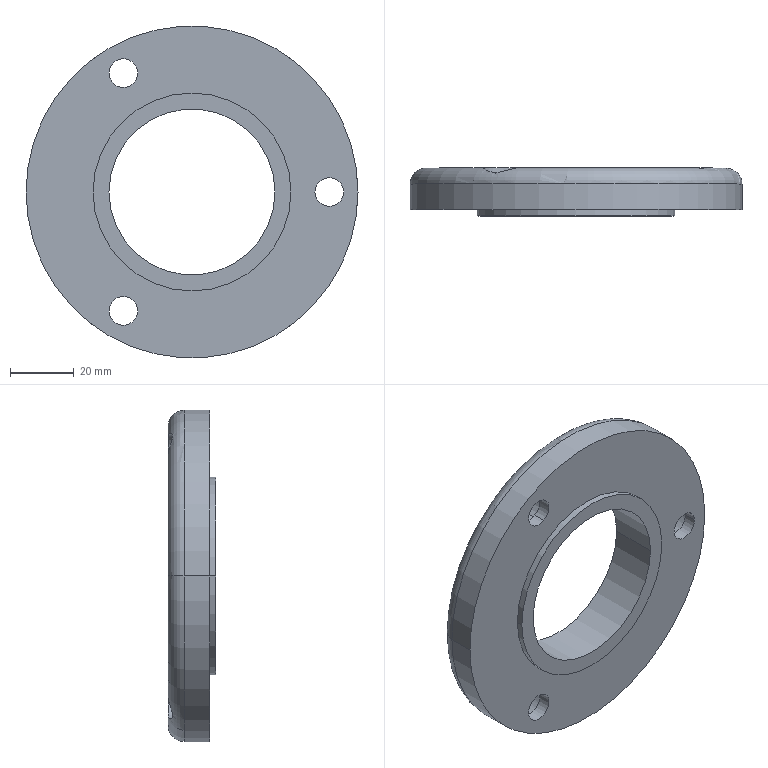Component | SolidWorks | 16-1 | 1 solid | 26 faces | box 104 x 15 x 104 mm | volume 77397 mm3 | cylinder 18 | plane 6 | torus 2 | commonest cylinder face diameters 15 x6 9 x6 52 x2 62 x2 104 x2
STEP:
#1=COLOUR_RGB('',0.7922,0.8196,0.9333);
#2=FILL_AREA_STYLE_COLOUR('',#1);
#3=FILL_AREA_STYLE('',(#2));
#4=SURFACE_STYLE_FILL_AREA(#3);
#5=SURFACE_SIDE_STYLE('',(#4));
#6=SURFACE_STYLE_USAGE(.BOTH.,#5);
#7=PRESENTATION_STYLE_ASSIGNMENT((#6));
#8=CARTESIAN_POINT('',(-1.85,-2.835,0.));
#9=VERTEX_POINT('',#8);
#10=CARTESIAN_POINT('',(-1.142,-2.835,1.456));
#11=VERTEX_POINT('',#10);
#12=CARTESIAN_POINT('',(0.,-2.835,-0.));
#13=DIRECTION('',(-0.,1.,0.));
#14=DIRECTION('',(1.,0.,0.));
#15=AXIS2_PLACEMENT_3D('',#12,#13,#14);
#16=CIRCLE('',#15,1.85);
#17=EDGE_CURVE('',#9,#11,#16,.T.);
#18=ORIENTED_EDGE('',*,*,#17,.F.);
#19=CARTESIAN_POINT('',(-2.047,-3.031,0.));
#20=VERTEX_POINT('',#19);
#21=CARTESIAN_POINT('',(-1.85,-3.031,0.));
#22=DIRECTION('',(0.,-0.,1.));
#23=DIRECTION('',(1.,0.,-0.));
#24=AXIS2_PLACEMENT_3D('',#21,#22,#23);
#25=CIRCLE('',#24,0.1969);
#26=EDGE_CURVE('',#9,#20,#25,.T.);
#27=ORIENTED_EDGE('',*,*,#26,.T.);
#28=CARTESIAN_POINT('',(2.047,-3.031,-0.));
#29=VERTEX_POINT('',#28);
#30=CARTESIAN_POINT('',(0.,-3.031,-0.));
#31=DIRECTION('',(0.,-1.,-0.));
#32=DIRECTION('',(1.,0.,-0.));
#33=AXIS2_PLACEMENT_3D('',#30,#31,#32);
#34=CIRCLE('',#33,2.047);
#35=EDGE_CURVE('',#29,#20,#34,.T.);
#36=ORIENTED_EDGE('',*,*,#35,.F.);
#37=CARTESIAN_POINT('',(1.988,-2.891,-0.));
#38=VERTEX_POINT('',#37);
#39=CARTESIAN_POINT('',(1.85,-3.031,-0.));
#40=DIRECTION('',(-0.,0.,-1.));
#41=DIRECTION('',(-1.,0.,0.));
#42=AXIS2_PLACEMENT_3D('',#39,#40,#41);
#43=CIRCLE('',#42,0.1969);
#44=EDGE_CURVE('',#38,#29,#43,.T.);
#45=ORIENTED_EDGE('',*,*,#44,.F.);
#46=CARTESIAN_POINT('',(1.832,-2.835,0.2605));
#47=VERTEX_POINT('',#46);
#48=CARTESIAN_POINT('',(1.832,-2.835,0.2605));
#49=CARTESIAN_POINT('',(1.856,-2.835,0.2476));
#50=CARTESIAN_POINT('',(1.878,-2.838,0.2318));
#51=CARTESIAN_POINT('',(1.907,-2.846,0.204));
#52=CARTESIAN_POINT('',(1.916,-2.849,0.1943));
#53=CARTESIAN_POINT('',(1.932,-2.856,0.1738));
#54=CARTESIAN_POINT('',(1.939,-2.859,0.1631));
#55=CARTESIAN_POINT('',(1.953,-2.866,0.1407));
#56=CARTESIAN_POINT('',(1.959,-2.87,0.1289));
#57=CARTESIAN_POINT('',(1.969,-2.877,0.1048));
#58=CARTESIAN_POINT('',(1.974,-2.88,0.09241));
#59=CARTESIAN_POINT('',(1.981,-2.885,0.06703));
#60=CARTESIAN_POINT('',(1.984,-2.887,0.054));
#61=CARTESIAN_POINT('',(1.987,-2.89,0.02716));
#62=CARTESIAN_POINT('',(1.988,-2.891,0.01351));
#63=CARTESIAN_POINT('',(1.988,-2.891,-0.));
#64=B_SPLINE_CURVE_WITH_KNOTS('',3,(#48,#49,#50,#51,#52,#53,#54,#55,#56,#57,#58,#59,#60,#61,#62,#63),.UNSPECIFIED.,.F.,.F.,(4,2,2,2,2,2,2,4),(0.,0.002055,0.003083,0.004111,0.005138,0.006166,0.007194,0.008222),.UNSPECIFIED.);
#65=EDGE_CURVE('',#47,#38,#64,.T.);
#66=ORIENTED_EDGE('',*,*,#65,.F.);
#67=CARTESIAN_POINT('',(-0.6904,-2.835,1.717));
#68=VERTEX_POINT('',#67);
#69=CARTESIAN_POINT('',(0.,-2.835,-0.));
#70=DIRECTION('',(-0.,1.,0.));
#71=DIRECTION('',(1.,0.,-0.));
#72=AXIS2_PLACEMENT_3D('',#69,#70,#71);
#73=CIRCLE('',#72,1.85);
#74=EDGE_CURVE('',#68,#47,#73,.T.);
#75=ORIENTED_EDGE('',*,*,#74,.F.);
#76=CARTESIAN_POINT('',(-0.9941,-2.891,1.722));
#77=VERTEX_POINT('',#76);
#78=CARTESIAN_POINT('',(-0.9941,-2.891,1.722));
#79=CARTESIAN_POINT('',(-0.9824,-2.891,1.729));
#80=CARTESIAN_POINT('',(-0.9703,-2.89,1.734));
#81=CARTESIAN_POINT('',(-0.9453,-2.887,1.745));
#82=CARTESIAN_POINT('',(-0.9325,-2.885,1.749));
#83=CARTESIAN_POINT('',(-0.894,-2.877,1.759));
#84=CARTESIAN_POINT('',(-0.8676,-2.87,1.762));
#85=CARTESIAN_POINT('',(-0.8286,-2.859,1.761));
#86=CARTESIAN_POINT('',(-0.8156,-2.856,1.76));
#87=CARTESIAN_POINT('',(-0.7896,-2.849,1.756));
#88=CARTESIAN_POINT('',(-0.7766,-2.846,1.753));
#89=CARTESIAN_POINT('',(-0.7512,-2.841,1.746));
#90=CARTESIAN_POINT('',(-0.7387,-2.839,1.741));
#91=CARTESIAN_POINT('',(-0.7141,-2.836,1.73));
#92=CARTESIAN_POINT('',(-0.702,-2.835,1.724));
#93=CARTESIAN_POINT('',(-0.6904,-2.835,1.717));
#94=B_SPLINE_CURVE_WITH_KNOTS('',3,(#78,#79,#80,#81,#82,#83,#84,#85,#86,#87,#88,#89,#90,#91,#92,#93),.UNSPECIFIED.,.F.,.F.,(4,2,2,2,2,2,2,4),(0.008222,0.009245,0.01027,0.01232,0.01334,0.01436,0.01539,0.01641),.UNSPECIFIED.);
#95=EDGE_CURVE('',#77,#68,#94,.T.);
#96=ORIENTED_EDGE('',*,*,#95,.F.);
#97=CARTESIAN_POINT('',(-1.142,-2.835,1.456));
#98=CARTESIAN_POINT('',(-1.142,-2.835,1.484));
#99=CARTESIAN_POINT('',(-1.14,-2.838,1.51));
#100=CARTESIAN_POINT('',(-1.13,-2.846,1.549));
#101=CARTESIAN_POINT('',(-1.126,-2.849,1.562));
#102=CARTESIAN_POINT('',(-1.117,-2.856,1.586));
#103=CARTESIAN_POINT('',(-1.111,-2.859,1.598));
#104=CARTESIAN_POINT('',(-1.098,-2.866,1.621));
#105=CARTESIAN_POINT('',(-1.091,-2.87,1.632));
#106=CARTESIAN_POINT('',(-1.075,-2.877,1.653));
#107=CARTESIAN_POINT('',(-1.067,-2.88,1.663));
#108=CARTESIAN_POINT('',(-1.048,-2.885,1.682));
#109=CARTESIAN_POINT('',(-1.039,-2.887,1.691));
#110=CARTESIAN_POINT('',(-1.017,-2.89,1.707));
#111=CARTESIAN_POINT('',(-1.006,-2.891,1.715));
#112=CARTESIAN_POINT('',(-0.9941,-2.891,1.722));
#113=B_SPLINE_CURVE_WITH_KNOTS('',3,(#97,#98,#99,#100,#101,#102,#103,#104,#105,#106,#107,#108,#109,#110,#111,#112),.UNSPECIFIED.,.F.,.F.,(4,2,2,2,2,2,2,4),(0.,0.002055,0.003083,0.004111,0.005138,0.006166,0.007194,0.008222),.UNSPECIFIED.);
#114=EDGE_CURVE('',#11,#77,#113,.T.);
#115=ORIENTED_EDGE('',*,*,#114,.F.);
#116=EDGE_LOOP('',(#18,#27,#36,#45,#66,#75,#96,#115));
#117=FACE_OUTER_BOUND('',#116,.T.);
#118=CARTESIAN_POINT('',(0.,-3.031,-0.));
#119=DIRECTION('',(0.,-1.,-0.));
#120=DIRECTION('',(1.,0.,-0.));
#121=AXIS2_PLACEMENT_3D('',#118,#119,#120);
#122=TOROIDAL_SURFACE('',#121,1.85,0.1969);
#123=ADVANCED_FACE('',(#117),#122,.T.);
#124=CARTESIAN_POINT('',(-0.9941,-3.189,1.722));
#125=VERTEX_POINT('',#124);
#126=CARTESIAN_POINT('',(-0.6988,-3.189,1.21));
#127=VERTEX_POINT('',#126);
#128=CARTESIAN_POINT('',(-0.8465,-3.189,1.466));
#129=DIRECTION('',(-0.,1.,0.));
#130=DIRECTION('',(0.5,0.,-0.866));
#131=AXIS2_PLACEMENT_3D('',#128,#129,#130);
#132=CIRCLE('',#131,0.2953);
#133=EDGE_CURVE('',#125,#127,#132,.T.);
#134=ORIENTED_EDGE('',*,*,#133,.F.);
#135=CARTESIAN_POINT('',(-0.9941,-2.835,1.722));
#136=DIRECTION('',(-0.,1.,0.));
#137=VECTOR('',#136,39.37);
#138=LINE('',#135,#137);
#139=EDGE_CURVE('',#125,#77,#138,.T.);
#140=ORIENTED_EDGE('',*,*,#139,.T.);
#141=ORIENTED_EDGE('',*,*,#95,.T.);
#142=CARTESIAN_POINT('',(-0.6988,-2.835,1.21));
#143=VERTEX_POINT('',#142);
#144=CARTESIAN_POINT('',(-0.8465,-2.835,1.466));
#145=DIRECTION('',(-0.,1.,0.));
#146=DIRECTION('',(0.5,0.,-0.866));
#147=AXIS2_PLACEMENT_3D('',#144,#145,#146);
#148=CIRCLE('',#147,0.2953);
#149=EDGE_CURVE('',#68,#143,#148,.T.);
#150=ORIENTED_EDGE('',*,*,#149,.T.);
#151=CARTESIAN_POINT('',(-0.6988,-2.835,1.21));
#152=DIRECTION('',(-0.,1.,0.));
#153=VECTOR('',#152,39.37);
#154=LINE('',#151,#153);
#155=EDGE_CURVE('',#127,#143,#154,.T.);
#156=ORIENTED_EDGE('',*,*,#155,.F.);
#157=EDGE_LOOP('',(#134,#140,#141,#150,#156));
#158=FACE_OUTER_BOUND('',#157,.T.);
#159=CARTESIAN_POINT('',(-0.8465,-2.835,1.466));
#160=DIRECTION('',(-0.,1.,0.));
#161=DIRECTION('',(0.5,0.,-0.866));
#162=AXIS2_PLACEMENT_3D('',#159,#160,#161);
#163=CYLINDRICAL_SURFACE('',#162,0.2953);
#164=ADVANCED_FACE('',(#158),#163,.F.);
#165=CARTESIAN_POINT('',(-0.7579,-3.346,1.313));
#166=VERTEX_POINT('',#165);
#167=CARTESIAN_POINT('',(-0.935,-3.346,1.62));
#168=VERTEX_POINT('',#167);
#169=CARTESIAN_POINT('',(-0.8465,-3.346,1.466));
#170=DIRECTION('',(0.,-1.,-0.));
#171=DIRECTION('',(-0.5,0.,0.866));
#172=AXIS2_PLACEMENT_3D('',#169,#170,#171);
#173=CIRCLE('',#172,0.1772);
#174=EDGE_CURVE('',#166,#168,#173,.T.);
#175=ORIENTED_EDGE('',*,*,#174,.T.);
#176=CARTESIAN_POINT('',(-0.935,-3.189,1.62));
#177=VERTEX_POINT('',#176);
#178=CARTESIAN_POINT('',(-0.935,-2.835,1.62));
#179=DIRECTION('',(-0.,1.,0.));
#180=VECTOR('',#179,39.37);
#181=LINE('',#178,#180);
#182=EDGE_CURVE('',#168,#177,#181,.T.);
#183=ORIENTED_EDGE('',*,*,#182,.T.);
#184=CARTESIAN_POINT('',(-0.7579,-3.189,1.313));
#185=VERTEX_POINT('',#184);
#186=CARTESIAN_POINT('',(-0.8465,-3.189,1.466));
#187=DIRECTION('',(-0.,1.,0.));
#188=DIRECTION('',(0.5,0.,-0.866));
#189=AXIS2_PLACEMENT_3D('',#186,#187,#188);
#190=CIRCLE('',#189,0.1772);
#191=EDGE_CURVE('',#177,#185,#190,.T.);
#192=ORIENTED_EDGE('',*,*,#191,.T.);
#193=CARTESIAN_POINT('',(-0.7579,-2.835,1.313));
#194=DIRECTION('',(-0.,1.,0.));
#195=VECTOR('',#194,39.37);
#196=LINE('',#193,#195);
#197=EDGE_CURVE('',#166,#185,#196,.T.);
#198=ORIENTED_EDGE('',*,*,#197,.F.);
#199=EDGE_LOOP('',(#175,#183,#192,#198));
#200=FACE_OUTER_BOUND('',#199,.T.);
#201=CARTESIAN_POINT('',(-0.8465,-2.835,1.466));
#202=DIRECTION('',(-0.,1.,0.));
#203=DIRECTION('',(0.5,0.,-0.866));
#204=AXIS2_PLACEMENT_3D('',#201,#202,#203);
#205=CYLINDRICAL_SURFACE('',#204,0.1772);
#206=ADVANCED_FACE('',(#200),#205,.F.);
#207=CARTESIAN_POINT('',(-0.9941,-3.189,-1.722));
#208=VERTEX_POINT('',#207);
#209=CARTESIAN_POINT('',(-0.6988,-3.189,-1.21));
#210=VERTEX_POINT('',#209);
#211=CARTESIAN_POINT('',(-0.8465,-3.189,-1.466));
#212=DIRECTION('',(-0.,1.,0.));
#213=DIRECTION('',(0.5,0.,0.866));
#214=AXIS2_PLACEMENT_3D('',#211,#212,#213);
#215=CIRCLE('',#214,0.2953);
#216=EDGE_CURVE('',#208,#210,#215,.T.);
#217=ORIENTED_EDGE('',*,*,#216,.F.);
#218=CARTESIAN_POINT('',(-0.9941,-2.891,-1.722));
#219=VERTEX_POINT('',#218);
#220=CARTESIAN_POINT('',(-0.9941,-2.835,-1.722));
#221=DIRECTION('',(-0.,1.,0.));
#222=VECTOR('',#221,39.37);
#223=LINE('',#220,#222);
#224=EDGE_CURVE('',#208,#219,#223,.T.);
#225=ORIENTED_EDGE('',*,*,#224,.T.);
#226=CARTESIAN_POINT('',(-1.142,-2.835,-1.456));
#227=VERTEX_POINT('',#226);
#228=CARTESIAN_POINT('',(-0.9941,-2.891,-1.722));
#229=CARTESIAN_POINT('',(-1.006,-2.891,-1.715));
#230=CARTESIAN_POINT('',(-1.017,-2.89,-1.708));
#231=CARTESIAN_POINT('',(-1.038,-2.887,-1.691));
#232=CARTESIAN_POINT('',(-1.048,-2.885,-1.682));
#233=CARTESIAN_POINT('',(-1.076,-2.877,-1.654));
#234=CARTESIAN_POINT('',(-1.092,-2.87,-1.632));
#235=CARTESIAN_POINT('',(-1.111,-2.859,-1.598));
#236=CARTESIAN_POINT('',(-1.116,-2.856,-1.586));
#237=CARTESIAN_POINT('',(-1.126,-2.849,-1.562));
#238=CARTESIAN_POINT('',(-1.13,-2.846,-1.549));
#239=CARTESIAN_POINT('',(-1.136,-2.841,-1.523));
#240=CARTESIAN_POINT('',(-1.139,-2.839,-1.51));
#241=CARTESIAN_POINT('',(-1.142,-2.836,-1.484));
#242=CARTESIAN_POINT('',(-1.142,-2.835,-1.47));
#243=CARTESIAN_POINT('',(-1.142,-2.835,-1.456));
#244=B_SPLINE_CURVE_WITH_KNOTS('',3,(#228,#229,#230,#231,#232,#233,#234,#235,#236,#237,#238,#239,#240,#241,#242,#243),.UNSPECIFIED.,.F.,.F.,(4,2,2,2,2,2,2,4),(0.008222,0.009245,0.01027,0.01232,0.01334,0.01436,0.01539,0.01641),.UNSPECIFIED.);
#245=EDGE_CURVE('',#219,#227,#244,.T.);
#246=ORIENTED_EDGE('',*,*,#245,.T.);
#247=CARTESIAN_POINT('',(-0.6988,-2.835,-1.21));
#248=VERTEX_POINT('',#247);
#249=CARTESIAN_POINT('',(-0.8465,-2.835,-1.466));
#250=DIRECTION('',(-0.,1.,0.));
#251=DIRECTION('',(0.5,0.,0.866));
#252=AXIS2_PLACEMENT_3D('',#249,#250,#251);
#253=CIRCLE('',#252,0.2953);
#254=EDGE_CURVE('',#227,#248,#253,.T.);
#255=ORIENTED_EDGE('',*,*,#254,.T.);
#256=CARTESIAN_POINT('',(-0.6988,-2.835,-1.21));
#257=DIRECTION('',(-0.,1.,0.));
#258=VECTOR('',#257,39.37);
#259=LINE('',#256,#258);
#260=EDGE_CURVE('',#210,#248,#259,.T.);
#261=ORIENTED_EDGE('',*,*,#260,.F.);
#262=EDGE_LOOP('',(#217,#225,#246,#255,#261));
#263=FACE_OUTER_BOUND('',#262,.T.);
#264=CARTESIAN_POINT('',(-0.8465,-2.835,-1.466));
#265=DIRECTION('',(-0.,1.,0.));
#266=DIRECTION('',(0.5,0.,0.866));
#267=AXIS2_PLACEMENT_3D('',#264,#265,#266);
#268=CYLINDRICAL_SURFACE('',#267,0.2953);
#269=ADVANCED_FACE('',(#263),#268,.F.);
#270=CARTESIAN_POINT('',(-0.7579,-3.346,-1.313));
#271=VERTEX_POINT('',#270);
#272=CARTESIAN_POINT('',(-0.935,-3.346,-1.62));
#273=VERTEX_POINT('',#272);
#274=CARTESIAN_POINT('',(-0.8465,-3.346,-1.466));
#275=DIRECTION('',(0.,-1.,-0.));
#276=DIRECTION('',(-0.5,0.,-0.866));
#277=AXIS2_PLACEMENT_3D('',#274,#275,#276);
#278=CIRCLE('',#277,0.1772);
#279=EDGE_CURVE('',#271,#273,#278,.T.);
#280=ORIENTED_EDGE('',*,*,#279,.T.);
#281=CARTESIAN_POINT('',(-0.935,-3.189,-1.62));
#282=VERTEX_POINT('',#281);
#283=CARTESIAN_POINT('',(-0.935,-2.835,-1.62));
#284=DIRECTION('',(-0.,1.,0.));
#285=VECTOR('',#284,39.37);
#286=LINE('',#283,#285);
#287=EDGE_CURVE('',#273,#282,#286,.T.);
#288=ORIENTED_EDGE('',*,*,#287,.T.);
#289=CARTESIAN_POINT('',(-0.7579,-3.189,-1.313));
#290=VERTEX_POINT('',#289);
#291=CARTESIAN_POINT('',(-0.8465,-3.189,-1.466));
#292=DIRECTION('',(-0.,1.,0.));
#293=DIRECTION('',(0.5,0.,0.866));
#294=AXIS2_PLACEMENT_3D('',#291,#292,#293);
#295=CIRCLE('',#294,0.1772);
#296=EDGE_CURVE('',#282,#290,#295,.T.);
#297=ORIENTED_EDGE('',*,*,#296,.T.);
#298=CARTESIAN_POINT('',(-0.7579,-2.835,-1.313));
#299=DIRECTION('',(-0.,1.,0.));
#300=VECTOR('',#299,39.37);
#301=LINE('',#298,#300);
#302=EDGE_CURVE('',#271,#290,#301,.T.);
#303=ORIENTED_EDGE('',*,*,#302,.F.);
#304=EDGE_LOOP('',(#280,#288,#297,#303));
#305=FACE_OUTER_BOUND('',#304,.T.);
#306=CARTESIAN_POINT('',(-0.8465,-2.835,-1.466));
#307=DIRECTION('',(-0.,1.,0.));
#308=DIRECTION('',(0.5,0.,0.866));
#309=AXIS2_PLACEMENT_3D('',#306,#307,#308);
#310=CYLINDRICAL_SURFACE('',#309,0.1772);
#311=ADVANCED_FACE('',(#305),#310,.F.);
#312=CARTESIAN_POINT('',(1.988,-3.189,-0.));
#313=VERTEX_POINT('',#312);
#314=CARTESIAN_POINT('',(1.398,-3.189,-0.));
#315=VERTEX_POINT('',#314);
#316=CARTESIAN_POINT('',(1.693,-3.189,-0.));
#317=DIRECTION('',(-0.,1.,0.));
#318=DIRECTION('',(-1.,0.,0.));
#319=AXIS2_PLACEMENT_3D('',#316,#317,#318);
#320=CIRCLE('',#319,0.2953);
#321=EDGE_CURVE('',#313,#315,#320,.T.);
#322=ORIENTED_EDGE('',*,*,#321,.F.);
#323=CARTESIAN_POINT('',(1.988,-2.835,-0.));
#324=DIRECTION('',(-0.,1.,0.));
#325=VECTOR('',#324,39.37);
#326=LINE('',#323,#325);
#327=EDGE_CURVE('',#313,#38,#326,.T.);
#328=ORIENTED_EDGE('',*,*,#327,.T.);
#329=CARTESIAN_POINT('',(1.832,-2.835,-0.2605));
#330=VERTEX_POINT('',#329);
#331=CARTESIAN_POINT('',(1.988,-2.891,-0.));
#332=CARTESIAN_POINT('',(1.988,-2.891,-0.01346));
#333=CARTESIAN_POINT('',(1.987,-2.89,-0.02689));
#334=CARTESIAN_POINT('',(1.984,-2.887,-0.0537));
#335=CARTESIAN_POINT('',(1.981,-2.885,-0.06684));
#336=CARTESIAN_POINT('',(1.97,-2.877,-0.1051));
#337=CARTESIAN_POINT('',(1.96,-2.87,-0.1295));
#338=CARTESIAN_POINT('',(1.939,-2.859,-0.163));
#339=CARTESIAN_POINT('',(1.932,-2.856,-0.1737));
#340=CARTESIAN_POINT('',(1.916,-2.849,-0.1943));
#341=CARTESIAN_POINT('',(1.907,-2.846,-0.2041));
#342=CARTESIAN_POINT('',(1.888,-2.841,-0.2224));
#343=CARTESIAN_POINT('',(1.877,-2.839,-0.231));
#344=CARTESIAN_POINT('',(1.856,-2.836,-0.2468));
#345=CARTESIAN_POINT('',(1.844,-2.835,-0.254));
#346=CARTESIAN_POINT('',(1.832,-2.835,-0.2605));
#347=B_SPLINE_CURVE_WITH_KNOTS('',3,(#331,#332,#333,#334,#335,#336,#337,#338,#339,#340,#341,#342,#343,#344,#345,#346),.UNSPECIFIED.,.F.,.F.,(4,2,2,2,2,2,2,4),(0.008222,0.009245,0.01027,0.01232,0.01334,0.01436,0.01539,0.01641),.UNSPECIFIED.);
#348=EDGE_CURVE('',#38,#330,#347,.T.);
#349=ORIENTED_EDGE('',*,*,#348,.T.);
#350=CARTESIAN_POINT('',(1.398,-2.835,-0.));
#351=VERTEX_POINT('',#350);
#352=CARTESIAN_POINT('',(1.693,-2.835,-0.));
#353=DIRECTION('',(-0.,1.,0.));
#354=DIRECTION('',(-1.,0.,0.));
#355=AXIS2_PLACEMENT_3D('',#352,#353,#354);
#356=CIRCLE('',#355,0.2953);
#357=EDGE_CURVE('',#330,#351,#356,.T.);
#358=ORIENTED_EDGE('',*,*,#357,.T.);
#359=CARTESIAN_POINT('',(1.398,-2.835,-0.));
#360=DIRECTION('',(-0.,1.,0.));
#361=VECTOR('',#360,39.37);
#362=LINE('',#359,#361);
#363=EDGE_CURVE('',#315,#351,#362,.T.);
#364=ORIENTED_EDGE('',*,*,#363,.F.);
#365=EDGE_LOOP('',(#322,#328,#349,#358,#364));
#366=FACE_OUTER_BOUND('',#365,.T.);
#367=CARTESIAN_POINT('',(1.693,-2.835,-0.));
#368=DIRECTION('',(-0.,1.,0.));
#369=DIRECTION('',(-1.,0.,0.));
#370=AXIS2_PLACEMENT_3D('',#367,#368,#369);
#371=CYLINDRICAL_SURFACE('',#370,0.2953);
#372=ADVANCED_FACE('',(#366),#371,.F.);
#373=CARTESIAN_POINT('',(1.516,-3.346,-0.));
#374=VERTEX_POINT('',#373);
#375=CARTESIAN_POINT('',(1.87,-3.346,-0.));
#376=VERTEX_POINT('',#375);
#377=CARTESIAN_POINT('',(1.693,-3.346,-0.));
#378=DIRECTION('',(0.,-1.,-0.));
#379=DIRECTION('',(1.,0.,-0.));
#380=AXIS2_PLACEMENT_3D('',#377,#378,#379);
#381=CIRCLE('',#380,0.1772);
#382=EDGE_CURVE('',#374,#376,#381,.T.);
#383=ORIENTED_EDGE('',*,*,#382,.T.);
#384=CARTESIAN_POINT('',(1.87,-3.189,-0.));
#385=VERTEX_POINT('',#384);
#386=CARTESIAN_POINT('',(1.87,-2.835,-0.));
#387=DIRECTION('',(-0.,1.,0.));
#388=VECTOR('',#387,39.37);
#389=LINE('',#386,#388);
#390=EDGE_CURVE('',#376,#385,#389,.T.);
#391=ORIENTED_EDGE('',*,*,#390,.T.);
#392=CARTESIAN_POINT('',(1.516,-3.189,-0.));
#393=VERTEX_POINT('',#392);
#394=CARTESIAN_POINT('',(1.693,-3.189,-0.));
#395=DIRECTION('',(-0.,1.,0.));
#396=DIRECTION('',(-1.,0.,0.));
#397=AXIS2_PLACEMENT_3D('',#394,#395,#396);
#398=CIRCLE('',#397,0.1772);
#399=EDGE_CURVE('',#385,#393,#398,.T.);
#400=ORIENTED_EDGE('',*,*,#399,.T.);
#401=CARTESIAN_POINT('',(1.516,-2.835,-0.));
#402=DIRECTION('',(-0.,1.,0.));
#403=VECTOR('',#402,39.37);
#404=LINE('',#401,#403);
#405=EDGE_CURVE('',#374,#393,#404,.T.);
#406=ORIENTED_EDGE('',*,*,#405,.F.);
#407=EDGE_LOOP('',(#383,#391,#400,#406));
#408=FACE_OUTER_BOUND('',#407,.T.);
#409=CARTESIAN_POINT('',(1.693,-2.835,-0.));
#410=DIRECTION('',(-0.,1.,0.));
#411=DIRECTION('',(-1.,0.,0.));
#412=AXIS2_PLACEMENT_3D('',#409,#410,#411);
#413=CYLINDRICAL_SURFACE('',#412,0.1772);
#414=ADVANCED_FACE('',(#408),#413,.F.);
#415=CARTESIAN_POINT('',(-1.024,-2.835,-0.));
#416=VERTEX_POINT('',#415);
#417=CARTESIAN_POINT('',(1.024,-2.835,-0.));
#418=VERTEX_POINT('',#417);
#419=CARTESIAN_POINT('',(0.,-2.835,-0.));
#420=DIRECTION('',(0.,-1.,-0.));
#421=DIRECTION('',(1.,0.,-0.));
#422=AXIS2_PLACEMENT_3D('',#419,#420,#421);
#423=CIRCLE('',#422,1.024);
#424=EDGE_CURVE('',#416,#418,#423,.T.);
#425=ORIENTED_EDGE('',*,*,#424,.F.);
#426=CARTESIAN_POINT('',(-1.024,-3.425,-0.));
#427=VERTEX_POINT('',#426);
#428=CARTESIAN_POINT('',(-1.024,-1.85,-0.));
#429=DIRECTION('',(0.,-1.,-0.));
#430=VECTOR('',#429,39.37);
#431=LINE('',#428,#430);
#432=EDGE_CURVE('',#416,#427,#431,.T.);
#433=ORIENTED_EDGE('',*,*,#432,.T.);
#434=CARTESIAN_POINT('',(1.024,-3.425,-0.));
#435=VERTEX_POINT('',#434);
#436=CARTESIAN_POINT('',(0.,-3.425,-0.));
#437=DIRECTION('',(0.,-1.,-0.));
#438=DIRECTION('',(1.,0.,-0.));
#439=AXIS2_PLACEMENT_3D('',#436,#437,#438);
#440=CIRCLE('',#439,1.024);
#441=EDGE_CURVE('',#427,#435,#440,.T.);
#442=ORIENTED_EDGE('',*,*,#441,.T.);
#443=CARTESIAN_POINT('',(1.024,-1.85,-0.));
#444=DIRECTION('',(0.,-1.,-0.));
#445=VECTOR('',#444,39.37);
#446=LINE('',#443,#445);
#447=EDGE_CURVE('',#418,#435,#446,.T.);
#448=ORIENTED_EDGE('',*,*,#447,.F.);
#449=EDGE_LOOP('',(#425,#433,#442,#448));
#450=FACE_OUTER_BOUND('',#449,.T.);
#451=CARTESIAN_POINT('',(0.,-1.85,-0.));
#452=DIRECTION('',(0.,-1.,-0.));
#453=DIRECTION('',(1.,0.,-0.));
#454=AXIS2_PLACEMENT_3D('',#451,#452,#453);
#455=CYLINDRICAL_SURFACE('',#454,1.024);
#456=ADVANCED_FACE('',(#450),#455,.F.);
#457=CARTESIAN_POINT('',(1.22,-3.425,-0.));
#458=VERTEX_POINT('',#457);
#459=CARTESIAN_POINT('',(-1.22,-3.425,-0.));
#460=VERTEX_POINT('',#459);
#461=CARTESIAN_POINT('',(0.,-3.425,-0.));
#462=DIRECTION('',(0.,-1.,-0.));
#463=DIRECTION('',(1.,0.,-0.));
#464=AXIS2_PLACEMENT_3D('',#461,#462,#463);
#465=CIRCLE('',#464,1.22);
#466=EDGE_CURVE('',#458,#460,#465,.T.);
#467=ORIENTED_EDGE('',*,*,#466,.F.);
#468=CARTESIAN_POINT('',(1.22,-3.346,-0.));
#469=VERTEX_POINT('',#468);
#470=CARTESIAN_POINT('',(1.22,-3.425,-0.));
#471=DIRECTION('',(-0.,1.,0.));
#472=VECTOR('',#471,39.37);
#473=LINE('',#470,#472);
#474=EDGE_CURVE('',#458,#469,#473,.T.);
#475=ORIENTED_EDGE('',*,*,#474,.T.);
#476=CARTESIAN_POINT('',(-1.22,-3.346,-0.));
#477=VERTEX_POINT('',#476);
#478=CARTESIAN_POINT('',(0.,-3.346,-0.));
#479=DIRECTION('',(0.,-1.,-0.));
#480=DIRECTION('',(1.,0.,-0.));
#481=AXIS2_PLACEMENT_3D('',#478,#479,#480);
#482=CIRCLE('',#481,1.22);
#483=EDGE_CURVE('',#469,#477,#482,.T.);
#484=ORIENTED_EDGE('',*,*,#483,.T.);
#485=CARTESIAN_POINT('',(-1.22,-3.425,-0.));
#486=DIRECTION('',(-0.,1.,0.));
#487=VECTOR('',#486,39.37);
#488=LINE('',#485,#487);
#489=EDGE_CURVE('',#460,#477,#488,.T.);
#490=ORIENTED_EDGE('',*,*,#489,.F.);
#491=EDGE_LOOP('',(#467,#475,#484,#490));
#492=FACE_OUTER_BOUND('',#491,.T.);
#493=CARTESIAN_POINT('',(0.,-3.425,-0.));
#494=DIRECTION('',(-0.,1.,0.));
#495=DIRECTION('',(-1.,0.,0.));
#496=AXIS2_PLACEMENT_3D('',#493,#494,#495);
#497=CYLINDRICAL_SURFACE('',#496,1.22);
#498=ADVANCED_FACE('',(#492),#497,.T.);
#499=CARTESIAN_POINT('',(2.047,-3.346,-0.));
#500=VERTEX_POINT('',#499);
#501=CARTESIAN_POINT('',(-2.047,-3.346,0.));
#502=VERTEX_POINT('',#501);
#503=CARTESIAN_POINT('',(0.,-3.346,-0.));
#504=DIRECTION('',(0.,-1.,-0.));
#505=DIRECTION('',(1.,0.,-0.));
#506=AXIS2_PLACEMENT_3D('',#503,#504,#505);
#507=CIRCLE('',#506,2.047);
#508=EDGE_CURVE('',#500,#502,#507,.T.);
#509=ORIENTED_EDGE('',*,*,#508,.F.);
#510=CARTESIAN_POINT('',(2.047,-3.346,-0.));
#511=DIRECTION('',(-0.,1.,0.));
#512=VECTOR('',#511,39.37);
#513=LINE('',#510,#512);
#514=EDGE_CURVE('',#500,#29,#513,.T.);
#515=ORIENTED_EDGE('',*,*,#514,.T.);
#516=ORIENTED_EDGE('',*,*,#35,.T.);
#517=CARTESIAN_POINT('',(-2.047,-3.346,0.));
#518=DIRECTION('',(-0.,1.,0.));
#519=VECTOR('',#518,39.37);
#520=LINE('',#517,#519);
#521=EDGE_CURVE('',#502,#20,#520,.T.);
#522=ORIENTED_EDGE('',*,*,#521,.F.);
#523=EDGE_LOOP('',(#509,#515,#516,#522));
#524=FACE_OUTER_BOUND('',#523,.T.);
#525=CARTESIAN_POINT('',(0.,-3.346,-0.));
#526=DIRECTION('',(-0.,1.,0.));
#527=DIRECTION('',(-1.,0.,0.));
#528=AXIS2_PLACEMENT_3D('',#525,#526,#527);
#529=CYLINDRICAL_SURFACE('',#528,2.047);
#530=ADVANCED_FACE('',(#524),#529,.T.);
#531=ORIENTED_EDGE('',*,*,#514,.F.);
#532=CARTESIAN_POINT('',(0.,-3.346,-0.));
#533=DIRECTION('',(0.,-1.,-0.));
#534=DIRECTION('',(1.,0.,-0.));
#535=AXIS2_PLACEMENT_3D('',#532,#533,#534);
#536=CIRCLE('',#535,2.047);
#537=EDGE_CURVE('',#502,#500,#536,.T.);
#538=ORIENTED_EDGE('',*,*,#537,.F.);
#539=ORIENTED_EDGE('',*,*,#521,.T.);
#540=CARTESIAN_POINT('',(0.,-3.031,-0.));
#541=DIRECTION('',(0.,-1.,-0.));
#542=DIRECTION('',(1.,0.,-0.));
#543=AXIS2_PLACEMENT_3D('',#540,#541,#542);
#544=CIRCLE('',#543,2.047);
#545=EDGE_CURVE('',#20,#29,#544,.T.);
#546=ORIENTED_EDGE('',*,*,#545,.T.);
#547=EDGE_LOOP('',(#531,#538,#539,#546));
#548=FACE_OUTER_BOUND('',#547,.T.);
#549=CARTESIAN_POINT('',(0.,-3.346,-0.));
#550=DIRECTION('',(-0.,1.,0.));
#551=DIRECTION('',(-1.,0.,0.));
#552=AXIS2_PLACEMENT_3D('',#549,#550,#551);
#553=CYLINDRICAL_SURFACE('',#552,2.047);
#554=ADVANCED_FACE('',(#548),#553,.T.);
#555=ORIENTED_EDGE('',*,*,#174,.F.);
#556=CARTESIAN_POINT('',(-0.8465,-3.346,1.466));
#557=DIRECTION('',(0.,-1.,-0.));
#558=DIRECTION('',(-0.5,0.,0.866));
#559=AXIS2_PLACEMENT_3D('',#556,#557,#558);
#560=CIRCLE('',#559,0.1772);
#561=EDGE_CURVE('',#168,#166,#560,.T.);
#562=ORIENTED_EDGE('',*,*,#561,.F.);
#563=EDGE_LOOP('',(#555,#562));
#564=FACE_BOUND('',#563,.T.);
#565=ORIENTED_EDGE('',*,*,#279,.F.);
#566=CARTESIAN_POINT('',(-0.8465,-3.346,-1.466));
#567=DIRECTION('',(0.,-1.,-0.));
#568=DIRECTION('',(-0.5,0.,-0.866));
#569=AXIS2_PLACEMENT_3D('',#566,#567,#568);
#570=CIRCLE('',#569,0.1772);
#571=EDGE_CURVE('',#273,#271,#570,.T.);
#572=ORIENTED_EDGE('',*,*,#571,.F.);
#573=EDGE_LOOP('',(#565,#572));
#574=FACE_BOUND('',#573,.T.);
#575=ORIENTED_EDGE('',*,*,#382,.F.);
#576=CARTESIAN_POINT('',(1.693,-3.346,-0.));
#577=DIRECTION('',(0.,-1.,-0.));
#578=DIRECTION('',(1.,0.,-0.));
#579=AXIS2_PLACEMENT_3D('',#576,#577,#578);
#580=CIRCLE('',#579,0.1772);
#581=EDGE_CURVE('',#376,#374,#580,.T.);
#582=ORIENTED_EDGE('',*,*,#581,.F.);
#583=EDGE_LOOP('',(#575,#582));
#584=FACE_BOUND('',#583,.T.);
#585=CARTESIAN_POINT('',(0.,-3.346,-0.));
#586=DIRECTION('',(0.,-1.,-0.));
#587=DIRECTION('',(1.,0.,-0.));
#588=AXIS2_PLACEMENT_3D('',#585,#586,#587);
#589=CIRCLE('',#588,1.22);
#590=EDGE_CURVE('',#477,#469,#589,.T.);
#591=ORIENTED_EDGE('',*,*,#590,.F.);
#592=ORIENTED_EDGE('',*,*,#483,.F.);
#593=EDGE_LOOP('',(#591,#592));
#594=FACE_BOUND('',#593,.T.);
#595=ORIENTED_EDGE('',*,*,#537,.T.);
#596=ORIENTED_EDGE('',*,*,#508,.T.);
#597=EDGE_LOOP('',(#595,#596));
#598=FACE_OUTER_BOUND('',#597,.T.);
#599=CARTESIAN_POINT('',(0.,-3.346,-0.));
#600=DIRECTION('',(0.,-1.,-0.));
#601=DIRECTION('',(1.,0.,-0.));
#602=AXIS2_PLACEMENT_3D('',#599,#600,#601);
#603=PLANE('',#602);
#604=ADVANCED_FACE('',(#564,#574,#584,#594,#598),#603,.T.);
#605=ORIENTED_EDGE('',*,*,#357,.F.);
#606=CARTESIAN_POINT('',(-0.6904,-2.835,-1.717));
#607=VERTEX_POINT('',#606);
#608=CARTESIAN_POINT('',(0.,-2.835,-0.));
#609=DIRECTION('',(-0.,1.,0.));
#610=DIRECTION('',(1.,0.,-0.));
#611=AXIS2_PLACEMENT_3D('',#608,#609,#610);
#612=CIRCLE('',#611,1.85);
#613=EDGE_CURVE('',#330,#607,#612,.T.);
#614=ORIENTED_EDGE('',*,*,#613,.T.);
#615=CARTESIAN_POINT('',(-0.8465,-2.835,-1.466));
#616=DIRECTION('',(-0.,1.,0.));
#617=DIRECTION('',(0.5,0.,0.866));
#618=AXIS2_PLACEMENT_3D('',#615,#616,#617);
#619=CIRCLE('',#618,0.2953);
#620=EDGE_CURVE('',#248,#607,#619,.T.);
#621=ORIENTED_EDGE('',*,*,#620,.F.);
#622=ORIENTED_EDGE('',*,*,#254,.F.);
#623=CARTESIAN_POINT('',(0.,-2.835,-0.));
#624=DIRECTION('',(-0.,1.,0.));
#625=DIRECTION('',(1.,0.,0.));
#626=AXIS2_PLACEMENT_3D('',#623,#624,#625);
#627=CIRCLE('',#626,1.85);
#628=EDGE_CURVE('',#227,#9,#627,.T.);
#629=ORIENTED_EDGE('',*,*,#628,.T.);
#630=ORIENTED_EDGE('',*,*,#17,.T.);
#631=CARTESIAN_POINT('',(-0.8465,-2.835,1.466));
#632=DIRECTION('',(-0.,1.,0.));
#633=DIRECTION('',(0.5,0.,-0.866));
#634=AXIS2_PLACEMENT_3D('',#631,#632,#633);
#635=CIRCLE('',#634,0.2953);
#636=EDGE_CURVE('',#143,#11,#635,.T.);
#637=ORIENTED_EDGE('',*,*,#636,.F.);
#638=ORIENTED_EDGE('',*,*,#149,.F.);
#639=ORIENTED_EDGE('',*,*,#74,.T.);
#640=CARTESIAN_POINT('',(1.693,-2.835,-0.));
#641=DIRECTION('',(-0.,1.,0.));
#642=DIRECTION('',(-1.,0.,0.));
#643=AXIS2_PLACEMENT_3D('',#640,#641,#642);
#644=CIRCLE('',#643,0.2953);
#645=EDGE_CURVE('',#351,#47,#644,.T.);
#646=ORIENTED_EDGE('',*,*,#645,.F.);
#647=EDGE_LOOP('',(#605,#614,#621,#622,#629,#630,#637,#638,#639,#646));
#648=FACE_OUTER_BOUND('',#647,.T.);
#649=CARTESIAN_POINT('',(0.,-2.835,-0.));
#650=DIRECTION('',(0.,-1.,-0.));
#651=DIRECTION('',(1.,0.,-0.));
#652=AXIS2_PLACEMENT_3D('',#649,#650,#651);
#653=CIRCLE('',#652,1.024);
#654=EDGE_CURVE('',#418,#416,#653,.T.);
#655=ORIENTED_EDGE('',*,*,#654,.T.);
#656=ORIENTED_EDGE('',*,*,#424,.T.);
#657=EDGE_LOOP('',(#655,#656));
#658=FACE_BOUND('',#657,.T.);
#659=CARTESIAN_POINT('',(0.,-2.835,-0.));
#660=DIRECTION('',(0.,-1.,-0.));
#661=DIRECTION('',(1.,0.,-0.));
#662=AXIS2_PLACEMENT_3D('',#659,#660,#661);
#663=PLANE('',#662);
#664=ADVANCED_FACE('',(#648,#658),#663,.F.);
#665=ORIENTED_EDGE('',*,*,#474,.F.);
#666=CARTESIAN_POINT('',(0.,-3.425,-0.));
#667=DIRECTION('',(0.,-1.,-0.));
#668=DIRECTION('',(1.,0.,-0.));
#669=AXIS2_PLACEMENT_3D('',#666,#667,#668);
#670=CIRCLE('',#669,1.22);
#671=EDGE_CURVE('',#460,#458,#670,.T.);
#672=ORIENTED_EDGE('',*,*,#671,.F.);
#673=ORIENTED_EDGE('',*,*,#489,.T.);
#674=ORIENTED_EDGE('',*,*,#590,.T.);
#675=EDGE_LOOP('',(#665,#672,#673,#674));
#676=FACE_OUTER_BOUND('',#675,.T.);
#677=CARTESIAN_POINT('',(0.,-3.425,-0.));
#678=DIRECTION('',(-0.,1.,0.));
#679=DIRECTION('',(-1.,0.,0.));
#680=AXIS2_PLACEMENT_3D('',#677,#678,#679);
#681=CYLINDRICAL_SURFACE('',#680,1.22);
#682=ADVANCED_FACE('',(#676),#681,.T.);
#683=CARTESIAN_POINT('',(0.,-3.425,-0.));
#684=DIRECTION('',(0.,-1.,-0.));
#685=DIRECTION('',(1.,0.,-0.));
#686=AXIS2_PLACEMENT_3D('',#683,#684,#685);
#687=CIRCLE('',#686,1.024);
#688=EDGE_CURVE('',#435,#427,#687,.T.);
#689=ORIENTED_EDGE('',*,*,#688,.F.);
#690=ORIENTED_EDGE('',*,*,#441,.F.);
#691=EDGE_LOOP('',(#689,#690));
#692=FACE_BOUND('',#691,.T.);
#693=ORIENTED_EDGE('',*,*,#671,.T.);
#694=ORIENTED_EDGE('',*,*,#466,.T.);
#695=EDGE_LOOP('',(#693,#694));
#696=FACE_OUTER_BOUND('',#695,.T.);
#697=CARTESIAN_POINT('',(0.,-3.425,-0.));
#698=DIRECTION('',(0.,-1.,-0.));
#699=DIRECTION('',(1.,0.,-0.));
#700=AXIS2_PLACEMENT_3D('',#697,#698,#699);
#701=PLANE('',#700);
#702=ADVANCED_FACE('',(#692,#696),#701,.T.);
#703=ORIENTED_EDGE('',*,*,#432,.F.);
#704=ORIENTED_EDGE('',*,*,#654,.F.);
#705=ORIENTED_EDGE('',*,*,#447,.T.);
#706=ORIENTED_EDGE('',*,*,#688,.T.);
#707=EDGE_LOOP('',(#703,#704,#705,#706));
#708=FACE_OUTER_BOUND('',#707,.T.);
#709=CARTESIAN_POINT('',(0.,-1.85,-0.));
#710=DIRECTION('',(0.,-1.,-0.));
#711=DIRECTION('',(1.,0.,-0.));
#712=AXIS2_PLACEMENT_3D('',#709,#710,#711);
#713=CYLINDRICAL_SURFACE('',#712,1.024);
#714=ADVANCED_FACE('',(#708),#713,.F.);
#715=ORIENTED_EDGE('',*,*,#390,.F.);
#716=ORIENTED_EDGE('',*,*,#581,.T.);
#717=ORIENTED_EDGE('',*,*,#405,.T.);
#718=CARTESIAN_POINT('',(1.693,-3.189,-0.));
#719=DIRECTION('',(-0.,1.,0.));
#720=DIRECTION('',(-1.,0.,0.));
#721=AXIS2_PLACEMENT_3D('',#718,#719,#720);
#722=CIRCLE('',#721,0.1772);
#723=EDGE_CURVE('',#393,#385,#722,.T.);
#724=ORIENTED_EDGE('',*,*,#723,.T.);
#725=EDGE_LOOP('',(#715,#716,#717,#724));
#726=FACE_OUTER_BOUND('',#725,.T.);
#727=CARTESIAN_POINT('',(1.693,-2.835,-0.));
#728=DIRECTION('',(-0.,1.,0.));
#729=DIRECTION('',(-1.,0.,0.));
#730=AXIS2_PLACEMENT_3D('',#727,#728,#729);
#731=CYLINDRICAL_SURFACE('',#730,0.1772);
#732=ADVANCED_FACE('',(#726),#731,.F.);
#733=ORIENTED_EDGE('',*,*,#723,.F.);
#734=ORIENTED_EDGE('',*,*,#399,.F.);
#735=EDGE_LOOP('',(#733,#734));
#736=FACE_BOUND('',#735,.T.);
#737=CARTESIAN_POINT('',(1.693,-3.189,-0.));
#738=DIRECTION('',(-0.,1.,0.));
#739=DIRECTION('',(-1.,0.,0.));
#740=AXIS2_PLACEMENT_3D('',#737,#738,#739);
#741=CIRCLE('',#740,0.2953);
#742=EDGE_CURVE('',#315,#313,#741,.T.);
#743=ORIENTED_EDGE('',*,*,#742,.T.);
#744=ORIENTED_EDGE('',*,*,#321,.T.);
#745=EDGE_LOOP('',(#743,#744));
#746=FACE_OUTER_BOUND('',#745,.T.);
#747=CARTESIAN_POINT('',(1.693,-3.189,0.1772));
#748=DIRECTION('',(0.,-1.,-0.));
#749=DIRECTION('',(1.,0.,-0.));
#750=AXIS2_PLACEMENT_3D('',#747,#748,#749);
#751=PLANE('',#750);
#752=ADVANCED_FACE('',(#736,#746),#751,.F.);
#753=ORIENTED_EDGE('',*,*,#327,.F.);
#754=ORIENTED_EDGE('',*,*,#742,.F.);
#755=ORIENTED_EDGE('',*,*,#363,.T.);
#756=ORIENTED_EDGE('',*,*,#645,.T.);
#757=ORIENTED_EDGE('',*,*,#65,.T.);
#758=EDGE_LOOP('',(#753,#754,#755,#756,#757));
#759=FACE_OUTER_BOUND('',#758,.T.);
#760=CARTESIAN_POINT('',(1.693,-2.835,-0.));
#761=DIRECTION('',(-0.,1.,0.));
#762=DIRECTION('',(-1.,0.,0.));
#763=AXIS2_PLACEMENT_3D('',#760,#761,#762);
#764=CYLINDRICAL_SURFACE('',#763,0.2953);
#765=ADVANCED_FACE('',(#759),#764,.F.);
#766=ORIENTED_EDGE('',*,*,#287,.F.);
#767=ORIENTED_EDGE('',*,*,#571,.T.);
#768=ORIENTED_EDGE('',*,*,#302,.T.);
#769=CARTESIAN_POINT('',(-0.8465,-3.189,-1.466));
#770=DIRECTION('',(-0.,1.,0.));
#771=DIRECTION('',(0.5,0.,0.866));
#772=AXIS2_PLACEMENT_3D('',#769,#770,#771);
#773=CIRCLE('',#772,0.1772);
#774=EDGE_CURVE('',#290,#282,#773,.T.);
#775=ORIENTED_EDGE('',*,*,#774,.T.);
#776=EDGE_LOOP('',(#766,#767,#768,#775));
#777=FACE_OUTER_BOUND('',#776,.T.);
#778=CARTESIAN_POINT('',(-0.8465,-2.835,-1.466));
#779=DIRECTION('',(-0.,1.,0.));
#780=DIRECTION('',(0.5,0.,0.866));
#781=AXIS2_PLACEMENT_3D('',#778,#779,#780);
#782=CYLINDRICAL_SURFACE('',#781,0.1772);
#783=ADVANCED_FACE('',(#777),#782,.F.);
#784=ORIENTED_EDGE('',*,*,#774,.F.);
#785=ORIENTED_EDGE('',*,*,#296,.F.);
#786=EDGE_LOOP('',(#784,#785));
#787=FACE_BOUND('',#786,.T.);
#788=CARTESIAN_POINT('',(-0.8465,-3.189,-1.466));
#789=DIRECTION('',(-0.,1.,0.));
#790=DIRECTION('',(0.5,0.,0.866));
#791=AXIS2_PLACEMENT_3D('',#788,#789,#790);
#792=CIRCLE('',#791,0.2953);
#793=EDGE_CURVE('',#210,#208,#792,.T.);
#794=ORIENTED_EDGE('',*,*,#793,.T.);
#795=ORIENTED_EDGE('',*,*,#216,.T.);
#796=EDGE_LOOP('',(#794,#795));
#797=FACE_OUTER_BOUND('',#796,.T.);
#798=CARTESIAN_POINT('',(-0.693,-3.189,-1.555));
#799=DIRECTION('',(0.,-1.,-0.));
#800=DIRECTION('',(-0.5,0.,-0.866));
#801=AXIS2_PLACEMENT_3D('',#798,#799,#800);
#802=PLANE('',#801);
#803=ADVANCED_FACE('',(#787,#797),#802,.F.);
#804=ORIENTED_EDGE('',*,*,#224,.F.);
#805=ORIENTED_EDGE('',*,*,#793,.F.);
#806=ORIENTED_EDGE('',*,*,#260,.T.);
#807=ORIENTED_EDGE('',*,*,#620,.T.);
#808=CARTESIAN_POINT('',(-0.6904,-2.835,-1.717));
#809=CARTESIAN_POINT('',(-0.7137,-2.835,-1.731));
#810=CARTESIAN_POINT('',(-0.7381,-2.838,-1.742));
#811=CARTESIAN_POINT('',(-0.7767,-2.846,-1.753));
#812=CARTESIAN_POINT('',(-0.7896,-2.849,-1.756));
#813=CARTESIAN_POINT('',(-0.8155,-2.856,-1.76));
#814=CARTESIAN_POINT('',(-0.8285,-2.859,-1.761));
#815=CARTESIAN_POINT('',(-0.8546,-2.866,-1.762));
#816=CARTESIAN_POINT('',(-0.8678,-2.87,-1.761));
#817=CARTESIAN_POINT('',(-0.8939,-2.877,-1.758));
#818=CARTESIAN_POINT('',(-0.9068,-2.88,-1.755));
#819=CARTESIAN_POINT('',(-0.9323,-2.885,-1.749));
#820=CARTESIAN_POINT('',(-0.945,-2.887,-1.745));
#821=CARTESIAN_POINT('',(-0.9701,-2.89,-1.735));
#822=CARTESIAN_POINT('',(-0.9824,-2.891,-1.729));
#823=CARTESIAN_POINT('',(-0.9941,-2.891,-1.722));
#824=B_SPLINE_CURVE_WITH_KNOTS('',3,(#808,#809,#810,#811,#812,#813,#814,#815,#816,#817,#818,#819,#820,#821,#822,#823),.UNSPECIFIED.,.F.,.F.,(4,2,2,2,2,2,2,4),(0.,0.002055,0.003083,0.004111,0.005138,0.006166,0.007194,0.008222),.UNSPECIFIED.);
#825=EDGE_CURVE('',#607,#219,#824,.T.);
#826=ORIENTED_EDGE('',*,*,#825,.T.);
#827=EDGE_LOOP('',(#804,#805,#806,#807,#826));
#828=FACE_OUTER_BOUND('',#827,.T.);
#829=CARTESIAN_POINT('',(-0.8465,-2.835,-1.466));
#830=DIRECTION('',(-0.,1.,0.));
#831=DIRECTION('',(0.5,0.,0.866));
#832=AXIS2_PLACEMENT_3D('',#829,#830,#831);
#833=CYLINDRICAL_SURFACE('',#832,0.2953);
#834=ADVANCED_FACE('',(#828),#833,.F.);
#835=ORIENTED_EDGE('',*,*,#182,.F.);
#836=ORIENTED_EDGE('',*,*,#561,.T.);
#837=ORIENTED_EDGE('',*,*,#197,.T.);
#838=CARTESIAN_POINT('',(-0.8465,-3.189,1.466));
#839=DIRECTION('',(-0.,1.,0.));
#840=DIRECTION('',(0.5,0.,-0.866));
#841=AXIS2_PLACEMENT_3D('',#838,#839,#840);
#842=CIRCLE('',#841,0.1772);
#843=EDGE_CURVE('',#185,#177,#842,.T.);
#844=ORIENTED_EDGE('',*,*,#843,.T.);
#845=EDGE_LOOP('',(#835,#836,#837,#844));
#846=FACE_OUTER_BOUND('',#845,.T.);
#847=CARTESIAN_POINT('',(-0.8465,-2.835,1.466));
#848=DIRECTION('',(-0.,1.,0.));
#849=DIRECTION('',(0.5,0.,-0.866));
#850=AXIS2_PLACEMENT_3D('',#847,#848,#849);
#851=CYLINDRICAL_SURFACE('',#850,0.1772);
#852=ADVANCED_FACE('',(#846),#851,.F.);
#853=ORIENTED_EDGE('',*,*,#843,.F.);
#854=ORIENTED_EDGE('',*,*,#191,.F.);
#855=EDGE_LOOP('',(#853,#854));
#856=FACE_BOUND('',#855,.T.);
#857=CARTESIAN_POINT('',(-0.8465,-3.189,1.466));
#858=DIRECTION('',(-0.,1.,0.));
#859=DIRECTION('',(0.5,0.,-0.866));
#860=AXIS2_PLACEMENT_3D('',#857,#858,#859);
#861=CIRCLE('',#860,0.2953);
#862=EDGE_CURVE('',#127,#125,#861,.T.);
#863=ORIENTED_EDGE('',*,*,#862,.T.);
#864=ORIENTED_EDGE('',*,*,#133,.T.);
#865=EDGE_LOOP('',(#863,#864));
#866=FACE_OUTER_BOUND('',#865,.T.);
#867=CARTESIAN_POINT('',(-0.9999,-3.189,1.378));
#868=DIRECTION('',(0.,-1.,-0.));
#869=DIRECTION('',(-0.5,-0.,0.866));
#870=AXIS2_PLACEMENT_3D('',#867,#868,#869);
#871=PLANE('',#870);
#872=ADVANCED_FACE('',(#856,#866),#871,.F.);
#873=ORIENTED_EDGE('',*,*,#139,.F.);
#874=ORIENTED_EDGE('',*,*,#862,.F.);
#875=ORIENTED_EDGE('',*,*,#155,.T.);
#876=ORIENTED_EDGE('',*,*,#636,.T.);
#877=ORIENTED_EDGE('',*,*,#114,.T.);
#878=EDGE_LOOP('',(#873,#874,#875,#876,#877));
#879=FACE_OUTER_BOUND('',#878,.T.);
#880=CARTESIAN_POINT('',(-0.8465,-2.835,1.466));
#881=DIRECTION('',(-0.,1.,0.));
#882=DIRECTION('',(0.5,0.,-0.866));
#883=AXIS2_PLACEMENT_3D('',#880,#881,#882);
#884=CYLINDRICAL_SURFACE('',#883,0.2953);
#885=ADVANCED_FACE('',(#879),#884,.F.);
#886=ORIENTED_EDGE('',*,*,#26,.F.);
#887=ORIENTED_EDGE('',*,*,#628,.F.);
#888=ORIENTED_EDGE('',*,*,#245,.F.);
#889=ORIENTED_EDGE('',*,*,#825,.F.);
#890=ORIENTED_EDGE('',*,*,#613,.F.);
#891=ORIENTED_EDGE('',*,*,#348,.F.);
#892=ORIENTED_EDGE('',*,*,#44,.T.);
#893=ORIENTED_EDGE('',*,*,#545,.F.);
#894=EDGE_LOOP('',(#886,#887,#888,#889,#890,#891,#892,#893));
#895=FACE_OUTER_BOUND('',#894,.T.);
#896=CARTESIAN_POINT('',(0.,-3.031,-0.));
#897=DIRECTION('',(0.,-1.,-0.));
#898=DIRECTION('',(1.,0.,-0.));
#899=AXIS2_PLACEMENT_3D('',#896,#897,#898);
#900=TOROIDAL_SURFACE('',#899,1.85,0.1969);
#901=ADVANCED_FACE('',(#895),#900,.T.);
#902=CLOSED_SHELL('',(#123,#164,#206,#269,#311,#372,#414,#456,#498,#530,#554,#604,#664,#682,#702,#714,#732,#752,#765,#783,#803,#834,#852,#872,#885,#901));
#903=MANIFOLD_SOLID_BREP('',#902);
#904=STYLED_ITEM('',(#7),#903);
#905=(LENGTH_UNIT()NAMED_UNIT(*)SI_UNIT($,.METRE.));
#906=LENGTH_MEASURE_WITH_UNIT(LENGTH_MEASURE(0.0254),#905);
#907=DIMENSIONAL_EXPONENTS(1.,0.,0.,0.,0.,0.,0.);
#908=(CONVERSION_BASED_UNIT('',#906)LENGTH_UNIT()NAMED_UNIT(#907));
#909=UNCERTAINTY_MEASURE_WITH_UNIT(LENGTH_MEASURE(0.00001),#908,'','');
#910=(NAMED_UNIT(*)PLANE_ANGLE_UNIT()SI_UNIT($,.RADIAN.));
#911=(NAMED_UNIT(*)SI_UNIT($,.STERADIAN.)SOLID_ANGLE_UNIT());
#912=(GEOMETRIC_REPRESENTATION_CONTEXT(3)GLOBAL_UNCERTAINTY_ASSIGNED_CONTEXT((#909))GLOBAL_UNIT_ASSIGNED_CONTEXT((#908,#910,#911))REPRESENTATION_CONTEXT('',''));
#913=MECHANICAL_DESIGN_GEOMETRIC_PRESENTATION_REPRESENTATION('',(#904),#912);
#914=PRESENTATION_LAYER_ASSIGNMENT('','',(#904));
#915=CARTESIAN_POINT('',(0.,0.,0.));
#916=DIRECTION('',(0.,0.,1.));
#917=DIRECTION('',(1.,0.,0.));
#918=AXIS2_PLACEMENT_3D('',#915,#916,#917);
#919=(LENGTH_UNIT()NAMED_UNIT(*)SI_UNIT($,.METRE.));
#920=LENGTH_MEASURE_WITH_UNIT(LENGTH_MEASURE(0.0254),#919);
#921=DIMENSIONAL_EXPONENTS(1.,0.,0.,0.,0.,0.,0.);
#922=(CONVERSION_BASED_UNIT('',#920)LENGTH_UNIT()NAMED_UNIT(#921));
#923=UNCERTAINTY_MEASURE_WITH_UNIT(LENGTH_MEASURE(0.00001),#922,'','');
#924=(NAMED_UNIT(*)PLANE_ANGLE_UNIT()SI_UNIT($,.RADIAN.));
#925=(NAMED_UNIT(*)SI_UNIT($,.STERADIAN.)SOLID_ANGLE_UNIT());
#926=(GEOMETRIC_REPRESENTATION_CONTEXT(3)GLOBAL_UNCERTAINTY_ASSIGNED_CONTEXT((#923))GLOBAL_UNIT_ASSIGNED_CONTEXT((#922,#924,#925))REPRESENTATION_CONTEXT('',''));
#927=ADVANCED_BREP_SHAPE_REPRESENTATION('',(#903,#918),#926);